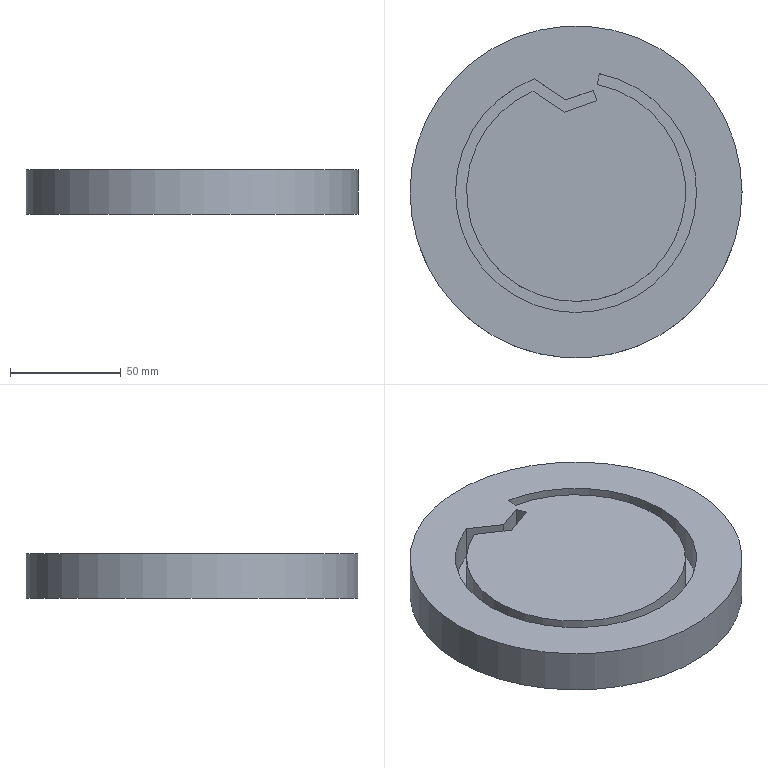CAM job | NX | mm | 3-axis | 1 set-up | 1 operations | part box 150 x 150 x 20
set-up 1
1. Planar Milling | Mill Mill5 MILL | PLANAR_MILL_1 | path 27814.643 mm | 10.179 min